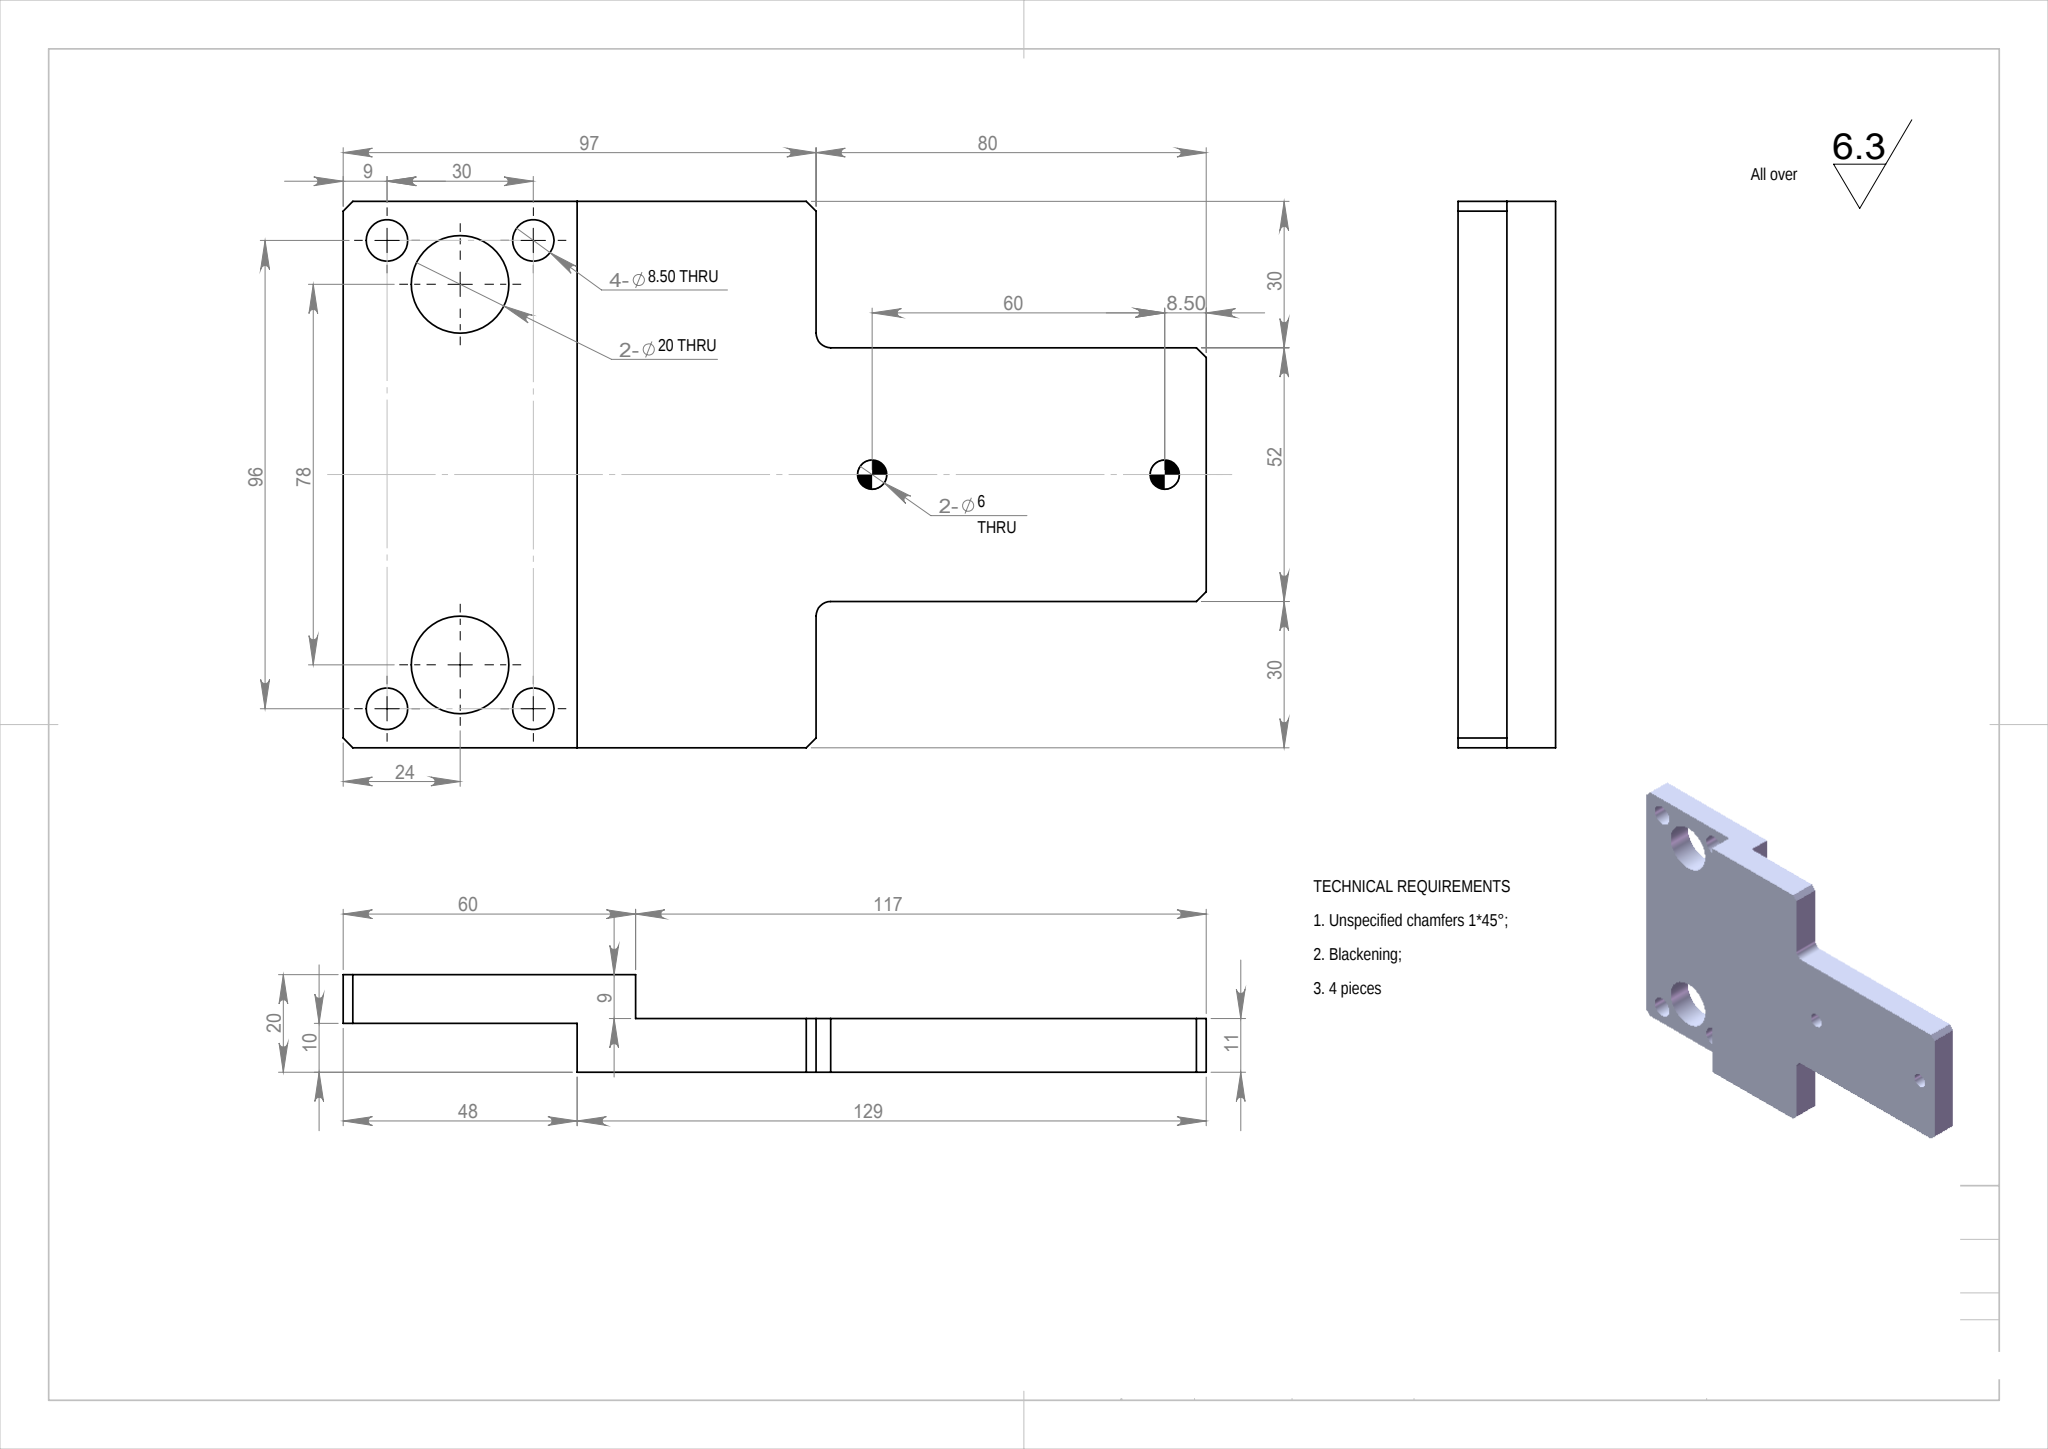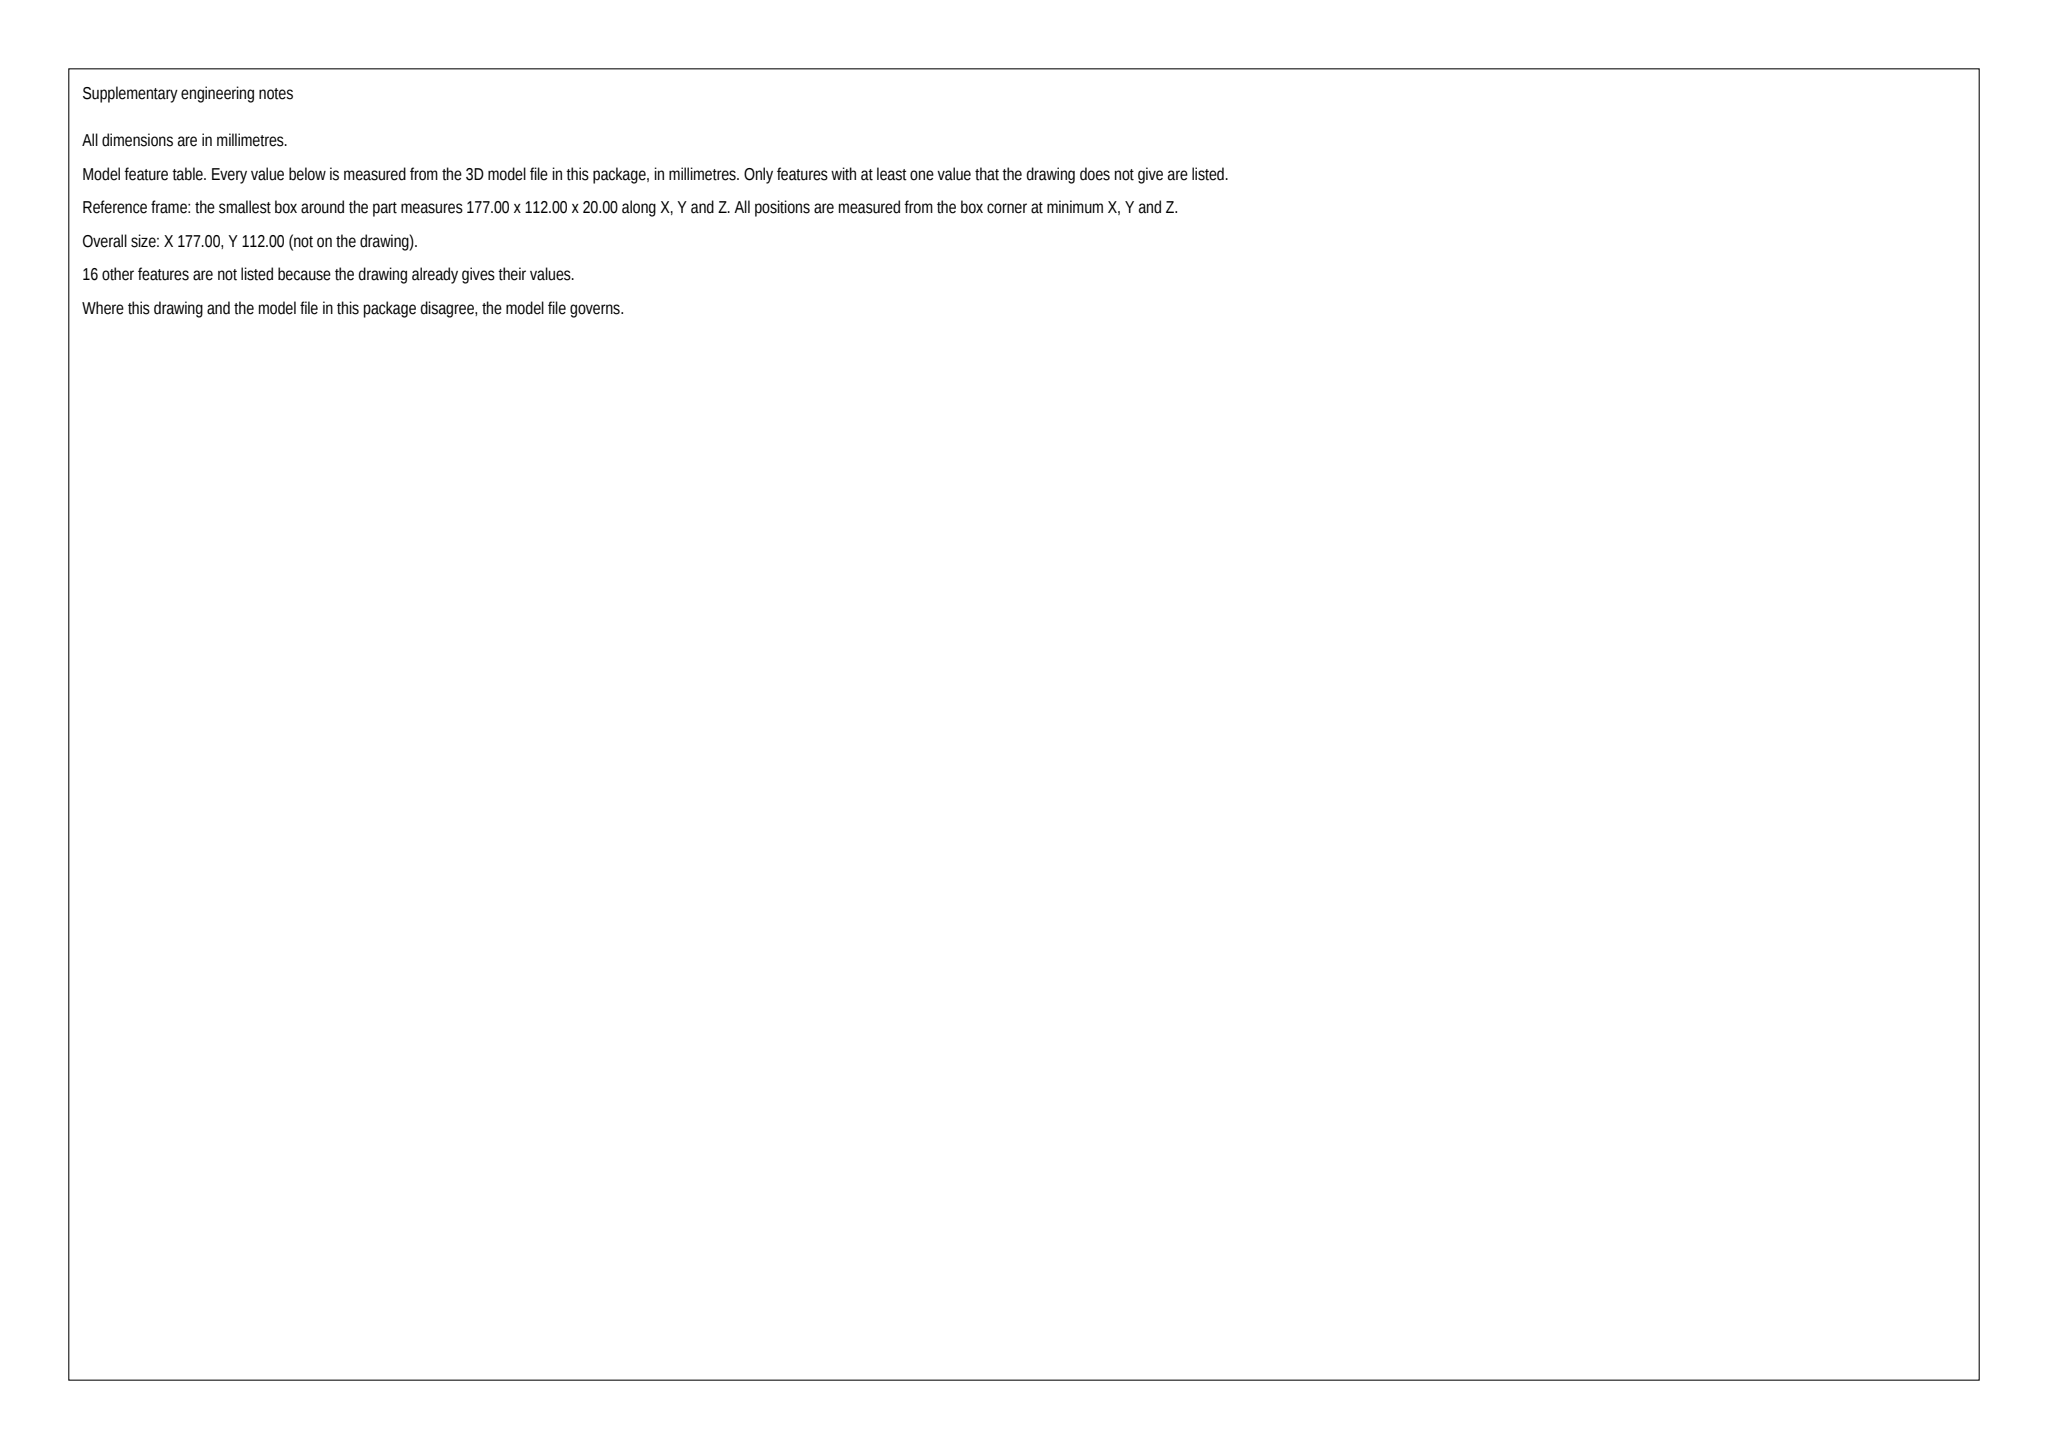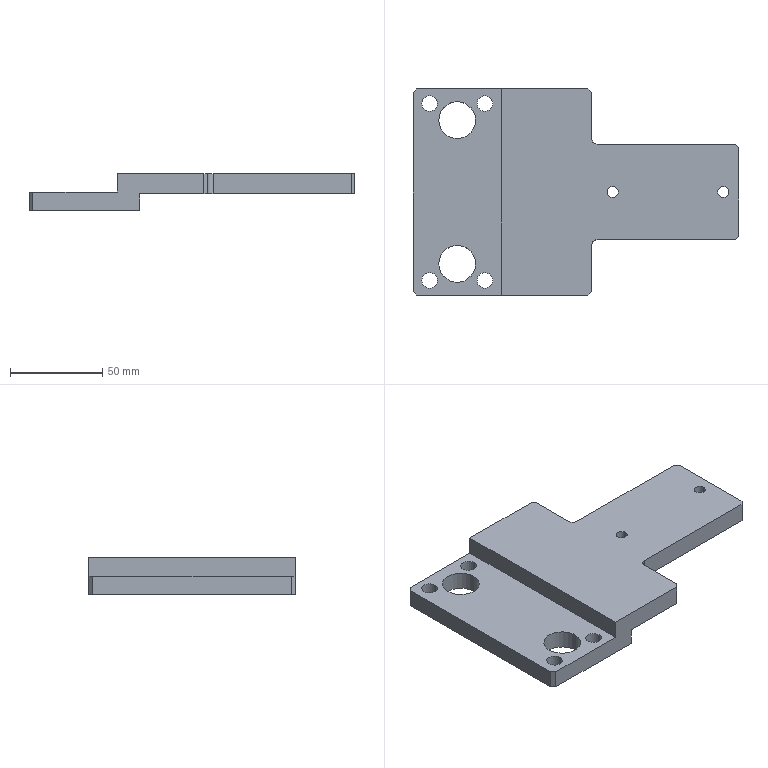Part | SolidWorks | mm | 1 solid | 38 faces | box 177 x 112 x 20 mm | volume 162723 mm3 | plane 20 | cylinder 18 | commonest cylinder face diameters 8.5 x8 6 x6 20 x4
build123d program:
from build123d import *

# Parameters (mm, degrees)
SKETCH1_W                 = 177
SKETCH1_H                 = 112
BOSS_EXTRUDE1_DEPTH       = 10
SKETCH3_W                 = 80
SKETCH3_H                 = 30
CUT_EXTRUDE2_DEPTH        = 107.622
FILLET1_R                 = 3
CHAMFER1_SIZE             = 2
SIZE_MM_DOWEL_PIN_HOLE1_D = 6
SKETCH10_W                = 117
SKETCH10_H                = 112
CUT_EXTRUDE3_DEPTH        = 9
SKETCH11_W                = 48
SKETCH11_H                = 112
CUT_EXTRUDE4_DEPTH        = 10
SKETCH12_R                = 10
CUT_EXTRUDE5_DEPTH        = 107.622
SKETCH13_R                = 4.25
CUT_EXTRUDE6_DEPTH        = 107.622


with BuildPart() as part:
    # Sketch1 → Boss-Extrude1 (new, symmetric)
    with BuildSketch(Plane.XY):
        Rectangle(SKETCH1_W, SKETCH1_H)
    extrude(amount=BOSS_EXTRUDE1_DEPTH, both=True)

    # Sketch3 → Cut-Extrude2 (cut, through all)
    with BuildSketch(Plane.XY.offset(10)):
        with Locations((48.5, 41)):
            Rectangle(SKETCH3_W, SKETCH3_H)
    cut_extrude2 = extrude(amount=-CUT_EXTRUDE2_DEPTH, mode=Mode.SUBTRACT)

    # Mirror1: Cut-Extrude2 across plane
    add(cut_extrude2.mirror(Plane.ZX), mode=Mode.SUBTRACT)

    # Fillet1
    fillet1_edges = [part.edges().sort_by_distance(p)[0] for p in [
        (8.5, 26, 0),
        (8.5, -26, 0),
    ]]
    fillet(fillet1_edges, radius=FILLET1_R)

    # Chamfer1
    chamfer1_edges = [part.edges().sort_by_distance(p)[0] for p in [
        (88.5, 26, 0),
        (8.5, 56, 0),
        (88.5, -26, 0),
        (8.5, -56, 0),
        (-88.5, -56, 0),
        (-88.5, 56, 0),
    ]]
    chamfer(chamfer1_edges, length=CHAMFER1_SIZE)

    # Size mm Dowel Pin Hole1 (through all)
    with Locations(Plane(origin=(0, 0, -10), x_dir=(-1, 0, 0), z_dir=(0, 0, -1))):
        with Locations((-20, 0), (-80, 0)):
            Hole(SIZE_MM_DOWEL_PIN_HOLE1_D / 2)

    # Sketch10 → Cut-Extrude3 (cut)
    with BuildSketch(Plane(origin=(0, 0, -10), x_dir=(-1, 0, 0), z_dir=(0, 0, -1))):
        with Locations((-30, 0)):
            Rectangle(SKETCH10_W, SKETCH10_H)
    extrude(amount=-CUT_EXTRUDE3_DEPTH, mode=Mode.SUBTRACT)

    # Sketch11 → Cut-Extrude4 (cut)
    with BuildSketch(Plane.XY.offset(10)):
        with Locations((-64.5, 0)):
            Rectangle(SKETCH11_W, SKETCH11_H)
    extrude(amount=-CUT_EXTRUDE4_DEPTH, mode=Mode.SUBTRACT)

    # Sketch12 → Cut-Extrude5 (cut, through all)
    with BuildSketch(Plane(origin=(0, 0, -10), x_dir=(-1, 0, 0), z_dir=(0, 0, -1))):
        with Locations((64.5, -39)):
            Circle(SKETCH12_R)
        with Locations((64.5, 39)):
            Circle(SKETCH12_R)
    extrude(amount=-CUT_EXTRUDE5_DEPTH, mode=Mode.SUBTRACT)

    # Sketch13 → Cut-Extrude6 (cut, through all)
    with BuildSketch(Plane(origin=(0, 0, -10), x_dir=(-1, 0, 0), z_dir=(0, 0, -1))):
        with Locations((49.5, 48)):
            Circle(SKETCH13_R)
        with Locations((79.5, 48)):
            Circle(SKETCH13_R)
        with Locations((79.5, -48)):
            Circle(SKETCH13_R)
        with Locations((49.5, -48)):
            Circle(SKETCH13_R)
    extrude(amount=-CUT_EXTRUDE6_DEPTH, mode=Mode.SUBTRACT)


solid = part.part